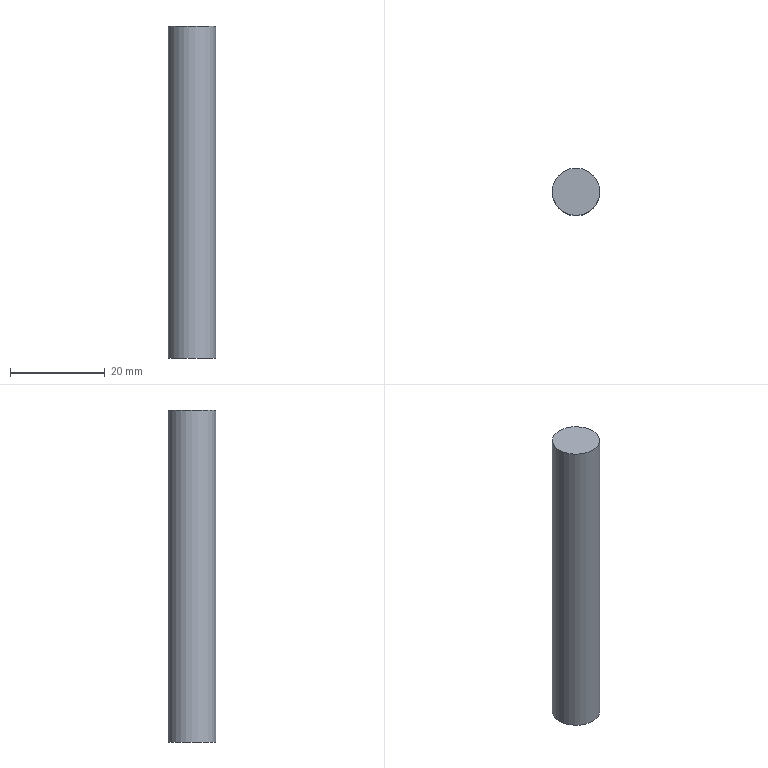Component | NX | A_STUD | 1 solid | 3 faces | box 10 x 10 x 70 mm | volume 5498 mm3 | plane 2 | cylinder 1 | commonest cylinder face diameters 10 x1
STEP:
#1=CARTESIAN_POINT('',(0.,0.,0.));
#2=DIRECTION('',(0.,0.,1.));
#3=DIRECTION('',(1.,0.,0.));
#4=AXIS2_PLACEMENT_3D('',#1,#2,#3);
#5=CARTESIAN_POINT('',(286.101,-0.,62.));
#6=VERTEX_POINT('',#5);
#7=CARTESIAN_POINT('',(291.101,-0.,62.));
#8=DIRECTION('',(0.,0.,-1.));
#9=DIRECTION('',(-1.,0.,0.));
#10=AXIS2_PLACEMENT_3D('',#7,#8,#9);
#11=CIRCLE('',#10,5.);
#12=CARTESIAN_POINT('',(291.101,-0.,62.));
#13=DIRECTION('',(0.,0.,1.));
#14=DIRECTION('',(-1.,0.,0.));
#15=AXIS2_PLACEMENT_3D('',#12,#13,#14);
#16=PLANE('',#15);
#17=CARTESIAN_POINT('',(5.,0.));
#18=CARTESIAN_POINT('',(5.,-8.66));
#19=CARTESIAN_POINT('',(-2.5,-4.33));
#20=CARTESIAN_POINT('',(-10.,-0.));
#21=CARTESIAN_POINT('',(-2.5,4.33));
#22=CARTESIAN_POINT('',(5.,8.66));
#23=CARTESIAN_POINT('',(5.,0.));
#24=(BOUNDED_CURVE()B_SPLINE_CURVE(2,(#17,#18,#19,#20,#21,#22,#23),.UNSPECIFIED.,.T.,.F.)B_SPLINE_CURVE_WITH_KNOTS((1,2,2,2,2,1),(-2.094,0.,2.094,4.189,6.283,8.378),.UNSPECIFIED.)CURVE()GEOMETRIC_REPRESENTATION_ITEM()RATIONAL_B_SPLINE_CURVE((1.,0.5,1.,0.5,1.,0.5,1.))REPRESENTATION_ITEM(''));
#25=(GEOMETRIC_REPRESENTATION_CONTEXT(2)PARAMETRIC_REPRESENTATION_CONTEXT()REPRESENTATION_CONTEXT('',''));
#26=DEFINITIONAL_REPRESENTATION('',(#24),#25);
#27=PCURVE('',#16,#26);
#28=CARTESIAN_POINT('',(291.101,-0.,-8.));
#29=DIRECTION('',(0.,0.,1.));
#30=DIRECTION('',(-1.,0.,0.));
#31=AXIS2_PLACEMENT_3D('',#28,#29,#30);
#32=CYLINDRICAL_SURFACE('',#31,5.);
#33=CARTESIAN_POINT('',(6.283,70.));
#34=DIRECTION('',(-1.,0.));
#35=VECTOR('',#34,1.);
#36=LINE('',#33,#35);
#37=(GEOMETRIC_REPRESENTATION_CONTEXT(2)PARAMETRIC_REPRESENTATION_CONTEXT()REPRESENTATION_CONTEXT('',''));
#38=DEFINITIONAL_REPRESENTATION('',(#36),#37);
#39=PCURVE('',#32,#38);
#40=SURFACE_CURVE('',#11,(#27,#39),.PCURVE_S1.);
#41=EDGE_CURVE('',#6,#6,#40,.T.);
#42=ORIENTED_EDGE('',*,*,#41,.F.);
#43=EDGE_LOOP('',(#42));
#44=FACE_BOUND('',#43,.T.);
#45=ADVANCED_FACE('',(#44),#16,.T.);
#46=CARTESIAN_POINT('',(286.101,-0.,-8.));
#47=VERTEX_POINT('',#46);
#48=CARTESIAN_POINT('',(291.101,-0.,-8.));
#49=DIRECTION('',(0.,0.,1.));
#50=DIRECTION('',(-1.,0.,0.));
#51=AXIS2_PLACEMENT_3D('',#48,#49,#50);
#52=CIRCLE('',#51,5.);
#53=CARTESIAN_POINT('',(291.101,-0.,-8.));
#54=DIRECTION('',(0.,0.,-1.));
#55=DIRECTION('',(1.,0.,0.));
#56=AXIS2_PLACEMENT_3D('',#53,#54,#55);
#57=PLANE('',#56);
#58=CARTESIAN_POINT('',(-5.,0.));
#59=CARTESIAN_POINT('',(-5.,8.66));
#60=CARTESIAN_POINT('',(2.5,4.33));
#61=CARTESIAN_POINT('',(10.,0.));
#62=CARTESIAN_POINT('',(2.5,-4.33));
#63=CARTESIAN_POINT('',(-5.,-8.66));
#64=CARTESIAN_POINT('',(-5.,0.));
#65=(BOUNDED_CURVE()B_SPLINE_CURVE(2,(#58,#59,#60,#61,#62,#63,#64),.UNSPECIFIED.,.T.,.F.)B_SPLINE_CURVE_WITH_KNOTS((1,2,2,2,2,1),(-2.094,0.,2.094,4.189,6.283,8.378),.UNSPECIFIED.)CURVE()GEOMETRIC_REPRESENTATION_ITEM()RATIONAL_B_SPLINE_CURVE((1.,0.5,1.,0.5,1.,0.5,1.))REPRESENTATION_ITEM(''));
#66=(GEOMETRIC_REPRESENTATION_CONTEXT(2)PARAMETRIC_REPRESENTATION_CONTEXT()REPRESENTATION_CONTEXT('',''));
#67=DEFINITIONAL_REPRESENTATION('',(#65),#66);
#68=PCURVE('',#57,#67);
#69=CARTESIAN_POINT('',(0.,0.));
#70=DIRECTION('',(1.,0.));
#71=VECTOR('',#70,1.);
#72=LINE('',#69,#71);
#73=(GEOMETRIC_REPRESENTATION_CONTEXT(2)PARAMETRIC_REPRESENTATION_CONTEXT()REPRESENTATION_CONTEXT('',''));
#74=DEFINITIONAL_REPRESENTATION('',(#72),#73);
#75=PCURVE('',#32,#74);
#76=SURFACE_CURVE('',#52,(#68,#75),.PCURVE_S1.);
#77=EDGE_CURVE('',#47,#47,#76,.T.);
#78=ORIENTED_EDGE('',*,*,#77,.F.);
#79=EDGE_LOOP('',(#78));
#80=FACE_BOUND('',#79,.T.);
#81=ADVANCED_FACE('',(#80),#57,.T.);
#82=ORIENTED_EDGE('',*,*,#41,.T.);
#83=CARTESIAN_POINT('',(286.101,-0.,-8.));
#84=CARTESIAN_POINT('',(286.101,-0.,62.));
#85=B_SPLINE_CURVE_WITH_KNOTS('',1,(#83,#84),.UNSPECIFIED.,.F.,.F.,(2,2),(0.,70.),.PIECEWISE_BEZIER_KNOTS.);
#86=CARTESIAN_POINT('',(0.,0.));
#87=DIRECTION('',(0.,1.));
#88=VECTOR('',#87,1.);
#89=LINE('',#86,#88);
#90=(GEOMETRIC_REPRESENTATION_CONTEXT(2)PARAMETRIC_REPRESENTATION_CONTEXT()REPRESENTATION_CONTEXT('',''));
#91=DEFINITIONAL_REPRESENTATION('',(#89),#90);
#92=PCURVE('',#32,#91);
#93=CARTESIAN_POINT('',(6.283,0.));
#94=DIRECTION('',(0.,1.));
#95=VECTOR('',#94,1.);
#96=LINE('',#93,#95);
#97=(GEOMETRIC_REPRESENTATION_CONTEXT(2)PARAMETRIC_REPRESENTATION_CONTEXT()REPRESENTATION_CONTEXT('',''));
#98=DEFINITIONAL_REPRESENTATION('',(#96),#97);
#99=PCURVE('',#32,#98);
#100=SEAM_CURVE('',#85,(#92,#99),.PCURVE_S1.);
#101=EDGE_CURVE('',#47,#6,#100,.T.);
#102=ORIENTED_EDGE('',*,*,#101,.F.);
#103=ORIENTED_EDGE('',*,*,#77,.T.);
#104=ORIENTED_EDGE('',*,*,#101,.T.);
#105=EDGE_LOOP('',(#82,#102,#103,#104));
#106=FACE_BOUND('',#105,.T.);
#107=ADVANCED_FACE('',(#106),#32,.T.);
#108=CLOSED_SHELL('',(#45,#81,#107));
#109=MANIFOLD_SOLID_BREP('',#108);
#110=(LENGTH_UNIT()NAMED_UNIT(*)SI_UNIT(.MILLI.,.METRE.));
#111=UNCERTAINTY_MEASURE_WITH_UNIT(LENGTH_MEASURE(0.00001),#110,'','');
#112=(NAMED_UNIT(*)PLANE_ANGLE_UNIT()SI_UNIT($,.RADIAN.));
#113=(NAMED_UNIT(*)SI_UNIT($,.STERADIAN.)SOLID_ANGLE_UNIT());
#114=(GEOMETRIC_REPRESENTATION_CONTEXT(3)GLOBAL_UNCERTAINTY_ASSIGNED_CONTEXT((#111))GLOBAL_UNIT_ASSIGNED_CONTEXT((#110,#112,#113))REPRESENTATION_CONTEXT('',''));
#115=ADVANCED_BREP_SHAPE_REPRESENTATION('',(#4,#109),#114);